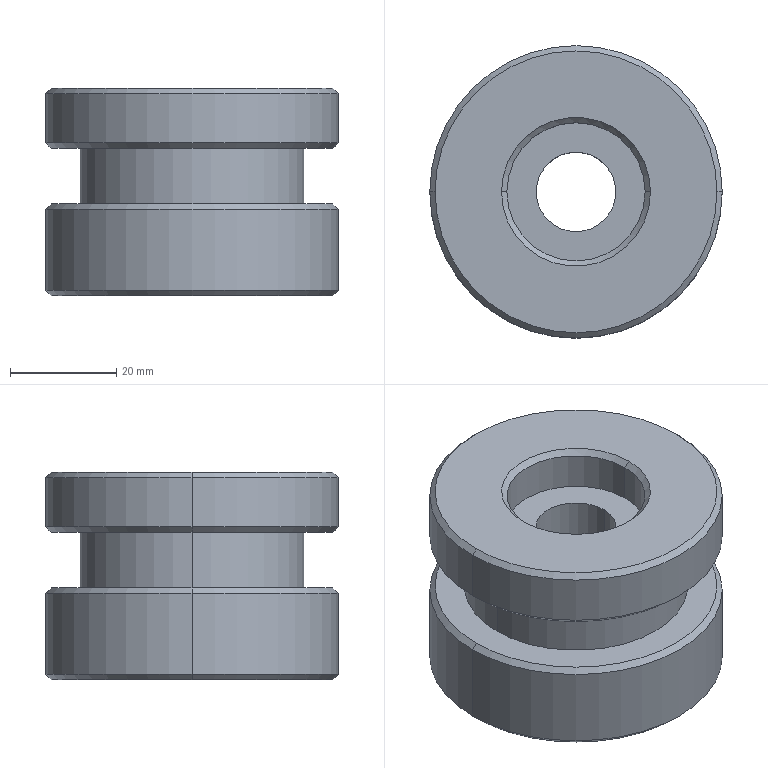Component | SolidWorks | 170423A4-PulleyAssembly-11_170423A4-Pulley1-1 | 1 solid | 30 faces | box 55 x 55 x 39 mm | volume 69274 mm3 | cone 12 | cylinder 12 | plane 6 | commonest cylinder face diameters 26 x4 55 x4 42 x2 15 x2
build123d program:
from build123d import *

# Parameters (mm, degrees)
SKETCH1_R           = 27.5
BOSS_EXTRUDE1_DEPTH = 19.5
SKETCH2_R           = 7.5
CUT_EXTRUDE1_DEPTH  = 56.077
SKETCH3_R           = 13
CUT_EXTRUDE2_DEPTH  = 8
CUT_EXTRUDE3_START  = -8
SKETCH4_R           = 13
CUT_EXTRUDE3_DEPTH  = 8
SKETCH5_W           = 6.5
SKETCH5_H           = 10.5
CHAMFER1_SIZE       = 1
CHAMFER2_SIZE       = 1


with BuildPart() as part:
    # Sketch1 → Boss-Extrude1 (new, symmetric)
    with BuildSketch(Plane.XY):
        Circle(SKETCH1_R)
    extrude(amount=BOSS_EXTRUDE1_DEPTH, both=True)

    # Sketch2 → Cut-Extrude1 (cut, through all)
    with BuildSketch(Plane.XY.offset(19.5)):
        Circle(SKETCH2_R)
    extrude(amount=-CUT_EXTRUDE1_DEPTH, mode=Mode.SUBTRACT)

    # Sketch3 → Cut-Extrude2 (cut)
    with BuildSketch(Plane.XY.offset(19.5)):
        Circle(SKETCH3_R)
    extrude(amount=-CUT_EXTRUDE2_DEPTH, mode=Mode.SUBTRACT)

    # Sketch4 → Cut-Extrude3 (cut)
    with BuildSketch(Plane(origin=(0, 0, -19.5), x_dir=(-1, 0, 0), z_dir=(0, 0, -1)).offset(CUT_EXTRUDE3_START)):
        with Locations(Location((0, 0, 0), (0, 0, 180))):
            Circle(SKETCH4_R)
    extrude(amount=CUT_EXTRUDE3_DEPTH, mode=Mode.SUBTRACT)

    # Sketch5 → Cut-Revolve1 (revolve, cut)
    with BuildSketch(Plane(origin=(0, 0, 0), x_dir=(1, 0, 0), z_dir=(0, 1, 0))):
        with Locations((-24.25, -3)):
            Rectangle(SKETCH5_W, SKETCH5_H)
    revolve(axis=Axis((0, 0, 0), (0, 0, 1)), mode=Mode.SUBTRACT)

    # Chamfer1
    chamfer1_edges = [part.edges().sort_by_distance(p)[0] for p in [
        (-27.5, 0, -19.5),
        (-27.5, 0, 8.25),
        (-27.5, 0, -2.25),
        (-27.5, 0, 19.5),
    ]]
    chamfer(chamfer1_edges, length=CHAMFER1_SIZE)

    # Chamfer2
    chamfer2_edges = [part.edges().sort_by_distance(p)[0] for p in [
        (-13, 0, 19.5),
        (-13, 0, -19.5),
    ]]
    chamfer(chamfer2_edges, length=CHAMFER2_SIZE)


solid = part.part

# Placed as in the assembly
solid = solid.moved(Location((139.754, -5.788, 441), (0, 0, 0)))
STEP:
#1=CARTESIAN_POINT('',(4.99,-0.2279,16.634));
#2=VERTEX_POINT('',#1);
#3=CARTESIAN_POINT('',(6.014,-0.2279,16.634));
#4=VERTEX_POINT('',#3);
#5=CARTESIAN_POINT('',(5.502,-0.2279,16.634));
#6=DIRECTION('',(0.,0.,-1.));
#7=DIRECTION('',(-1.,0.,0.));
#8=AXIS2_PLACEMENT_3D('',#5,#6,#7);
#9=CIRCLE('',#8,0.5118);
#10=EDGE_CURVE('',#2,#4,#9,.T.);
#11=ORIENTED_EDGE('',*,*,#10,.F.);
#12=CARTESIAN_POINT('',(4.951,-0.2279,16.594));
#13=VERTEX_POINT('',#12);
#14=CARTESIAN_POINT('',(4.99,-0.2279,16.634));
#15=DIRECTION('',(-0.7071,-0.,-0.7071));
#16=VECTOR('',#15,39.37);
#17=LINE('',#14,#16);
#18=EDGE_CURVE('',#2,#13,#17,.T.);
#19=ORIENTED_EDGE('',*,*,#18,.T.);
#20=CARTESIAN_POINT('',(6.053,-0.2279,16.594));
#21=VERTEX_POINT('',#20);
#22=CARTESIAN_POINT('',(5.502,-0.2279,16.594));
#23=DIRECTION('',(0.,0.,1.));
#24=DIRECTION('',(-1.,0.,0.));
#25=AXIS2_PLACEMENT_3D('',#22,#23,#24);
#26=CIRCLE('',#25,0.5512);
#27=EDGE_CURVE('',#21,#13,#26,.T.);
#28=ORIENTED_EDGE('',*,*,#27,.F.);
#29=CARTESIAN_POINT('',(6.014,-0.2279,16.634));
#30=DIRECTION('',(0.7071,0.,-0.7071));
#31=VECTOR('',#30,39.37);
#32=LINE('',#29,#31);
#33=EDGE_CURVE('',#4,#21,#32,.T.);
#34=ORIENTED_EDGE('',*,*,#33,.F.);
#35=EDGE_LOOP('',(#11,#19,#28,#34));
#36=FACE_OUTER_BOUND('',#35,.T.);
#37=CARTESIAN_POINT('',(5.502,-0.2279,16.634));
#38=DIRECTION('',(0.,0.,-1.));
#39=DIRECTION('',(1.,0.,0.));
#40=AXIS2_PLACEMENT_3D('',#37,#38,#39);
#41=CONICAL_SURFACE('',#40,0.5118,0.7854);
#42=ADVANCED_FACE('',(#36),#41,.F.);
#43=CARTESIAN_POINT('',(6.014,-0.2279,18.091));
#44=VERTEX_POINT('',#43);
#45=CARTESIAN_POINT('',(4.99,-0.2279,18.091));
#46=VERTEX_POINT('',#45);
#47=CARTESIAN_POINT('',(5.502,-0.2279,18.091));
#48=DIRECTION('',(0.,0.,1.));
#49=DIRECTION('',(-1.,0.,0.));
#50=AXIS2_PLACEMENT_3D('',#47,#48,#49);
#51=CIRCLE('',#50,0.5118);
#52=EDGE_CURVE('',#44,#46,#51,.T.);
#53=ORIENTED_EDGE('',*,*,#52,.F.);
#54=CARTESIAN_POINT('',(6.053,-0.2279,18.13));
#55=VERTEX_POINT('',#54);
#56=CARTESIAN_POINT('',(6.014,-0.2279,18.091));
#57=DIRECTION('',(0.7071,-0.,0.7071));
#58=VECTOR('',#57,39.37);
#59=LINE('',#56,#58);
#60=EDGE_CURVE('',#44,#55,#59,.T.);
#61=ORIENTED_EDGE('',*,*,#60,.T.);
#62=CARTESIAN_POINT('',(4.951,-0.2279,18.13));
#63=VERTEX_POINT('',#62);
#64=CARTESIAN_POINT('',(5.502,-0.2279,18.13));
#65=DIRECTION('',(0.,0.,-1.));
#66=DIRECTION('',(-1.,0.,0.));
#67=AXIS2_PLACEMENT_3D('',#64,#65,#66);
#68=CIRCLE('',#67,0.5512);
#69=EDGE_CURVE('',#63,#55,#68,.T.);
#70=ORIENTED_EDGE('',*,*,#69,.F.);
#71=CARTESIAN_POINT('',(4.99,-0.2279,18.091));
#72=DIRECTION('',(-0.7071,0.,0.7071));
#73=VECTOR('',#72,39.37);
#74=LINE('',#71,#73);
#75=EDGE_CURVE('',#46,#63,#74,.T.);
#76=ORIENTED_EDGE('',*,*,#75,.F.);
#77=EDGE_LOOP('',(#53,#61,#70,#76));
#78=FACE_OUTER_BOUND('',#77,.T.);
#79=CARTESIAN_POINT('',(5.502,-0.2279,18.091));
#80=DIRECTION('',(0.,0.,1.));
#81=DIRECTION('',(-1.,0.,0.));
#82=AXIS2_PLACEMENT_3D('',#79,#80,#81);
#83=CONICAL_SURFACE('',#82,0.5118,0.7854);
#84=ADVANCED_FACE('',(#78),#83,.F.);
#85=CARTESIAN_POINT('',(4.459,-0.2279,18.13));
#86=VERTEX_POINT('',#85);
#87=CARTESIAN_POINT('',(6.545,-0.2279,18.13));
#88=VERTEX_POINT('',#87);
#89=CARTESIAN_POINT('',(5.502,-0.2279,18.13));
#90=DIRECTION('',(0.,0.,1.));
#91=DIRECTION('',(-1.,0.,0.));
#92=AXIS2_PLACEMENT_3D('',#89,#90,#91);
#93=CIRCLE('',#92,1.043);
#94=EDGE_CURVE('',#86,#88,#93,.T.);
#95=ORIENTED_EDGE('',*,*,#94,.F.);
#96=CARTESIAN_POINT('',(4.419,-0.2279,18.091));
#97=VERTEX_POINT('',#96);
#98=CARTESIAN_POINT('',(4.459,-0.2279,18.13));
#99=DIRECTION('',(-0.7071,-0.,-0.7071));
#100=VECTOR('',#99,39.37);
#101=LINE('',#98,#100);
#102=EDGE_CURVE('',#86,#97,#101,.T.);
#103=ORIENTED_EDGE('',*,*,#102,.T.);
#104=CARTESIAN_POINT('',(6.585,-0.2279,18.091));
#105=VERTEX_POINT('',#104);
#106=CARTESIAN_POINT('',(5.502,-0.2279,18.091));
#107=DIRECTION('',(0.,0.,-1.));
#108=DIRECTION('',(-1.,0.,0.));
#109=AXIS2_PLACEMENT_3D('',#106,#107,#108);
#110=CIRCLE('',#109,1.083);
#111=EDGE_CURVE('',#105,#97,#110,.T.);
#112=ORIENTED_EDGE('',*,*,#111,.F.);
#113=CARTESIAN_POINT('',(6.545,-0.2279,18.13));
#114=DIRECTION('',(0.7071,0.,-0.7071));
#115=VECTOR('',#114,39.37);
#116=LINE('',#113,#115);
#117=EDGE_CURVE('',#88,#105,#116,.T.);
#118=ORIENTED_EDGE('',*,*,#117,.F.);
#119=EDGE_LOOP('',(#95,#103,#112,#118));
#120=FACE_OUTER_BOUND('',#119,.T.);
#121=CARTESIAN_POINT('',(5.502,-0.2279,18.13));
#122=DIRECTION('',(0.,0.,-1.));
#123=DIRECTION('',(1.,0.,0.));
#124=AXIS2_PLACEMENT_3D('',#121,#122,#123);
#125=CONICAL_SURFACE('',#124,1.043,0.7854);
#126=ADVANCED_FACE('',(#120),#125,.T.);
#127=CARTESIAN_POINT('',(6.545,-0.2279,17.687));
#128=VERTEX_POINT('',#127);
#129=CARTESIAN_POINT('',(4.459,-0.2279,17.687));
#130=VERTEX_POINT('',#129);
#131=CARTESIAN_POINT('',(5.502,-0.2279,17.687));
#132=DIRECTION('',(0.,0.,-1.));
#133=DIRECTION('',(-1.,0.,0.));
#134=AXIS2_PLACEMENT_3D('',#131,#132,#133);
#135=CIRCLE('',#134,1.043);
#136=EDGE_CURVE('',#128,#130,#135,.T.);
#137=ORIENTED_EDGE('',*,*,#136,.F.);
#138=CARTESIAN_POINT('',(6.585,-0.2279,17.726));
#139=VERTEX_POINT('',#138);
#140=CARTESIAN_POINT('',(6.545,-0.2279,17.687));
#141=DIRECTION('',(0.7071,-0.,0.7071));
#142=VECTOR('',#141,39.37);
#143=LINE('',#140,#142);
#144=EDGE_CURVE('',#128,#139,#143,.T.);
#145=ORIENTED_EDGE('',*,*,#144,.T.);
#146=CARTESIAN_POINT('',(4.419,-0.2279,17.726));
#147=VERTEX_POINT('',#146);
#148=CARTESIAN_POINT('',(5.502,-0.2279,17.726));
#149=DIRECTION('',(0.,0.,1.));
#150=DIRECTION('',(-1.,0.,0.));
#151=AXIS2_PLACEMENT_3D('',#148,#149,#150);
#152=CIRCLE('',#151,1.083);
#153=EDGE_CURVE('',#147,#139,#152,.T.);
#154=ORIENTED_EDGE('',*,*,#153,.F.);
#155=CARTESIAN_POINT('',(4.459,-0.2279,17.687));
#156=DIRECTION('',(-0.7071,0.,0.7071));
#157=VECTOR('',#156,39.37);
#158=LINE('',#155,#157);
#159=EDGE_CURVE('',#130,#147,#158,.T.);
#160=ORIENTED_EDGE('',*,*,#159,.F.);
#161=EDGE_LOOP('',(#137,#145,#154,#160));
#162=FACE_OUTER_BOUND('',#161,.T.);
#163=CARTESIAN_POINT('',(5.502,-0.2279,17.687));
#164=DIRECTION('',(0.,0.,1.));
#165=DIRECTION('',(-1.,0.,0.));
#166=AXIS2_PLACEMENT_3D('',#163,#164,#165);
#167=CONICAL_SURFACE('',#166,1.043,0.7854);
#168=ADVANCED_FACE('',(#162),#167,.T.);
#169=CARTESIAN_POINT('',(4.459,-0.2279,17.274));
#170=VERTEX_POINT('',#169);
#171=CARTESIAN_POINT('',(6.545,-0.2279,17.274));
#172=VERTEX_POINT('',#171);
#173=CARTESIAN_POINT('',(5.502,-0.2279,17.274));
#174=DIRECTION('',(-0.,0.,1.));
#175=DIRECTION('',(1.,0.,0.));
#176=AXIS2_PLACEMENT_3D('',#173,#174,#175);
#177=CIRCLE('',#176,1.043);
#178=EDGE_CURVE('',#170,#172,#177,.T.);
#179=ORIENTED_EDGE('',*,*,#178,.F.);
#180=CARTESIAN_POINT('',(4.419,-0.2279,17.234));
#181=VERTEX_POINT('',#180);
#182=CARTESIAN_POINT('',(4.419,-0.2279,17.234));
#183=DIRECTION('',(-0.7071,-0.,-0.7071));
#184=VECTOR('',#183,39.37);
#185=LINE('',#182,#184);
#186=EDGE_CURVE('',#170,#181,#185,.T.);
#187=ORIENTED_EDGE('',*,*,#186,.T.);
#188=CARTESIAN_POINT('',(6.585,-0.2279,17.234));
#189=VERTEX_POINT('',#188);
#190=CARTESIAN_POINT('',(5.502,-0.2279,17.234));
#191=DIRECTION('',(0.,0.,-1.));
#192=DIRECTION('',(1.,0.,0.));
#193=AXIS2_PLACEMENT_3D('',#190,#191,#192);
#194=CIRCLE('',#193,1.083);
#195=EDGE_CURVE('',#189,#181,#194,.T.);
#196=ORIENTED_EDGE('',*,*,#195,.F.);
#197=CARTESIAN_POINT('',(6.585,-0.2279,17.234));
#198=DIRECTION('',(0.7071,0.,-0.7071));
#199=VECTOR('',#198,39.37);
#200=LINE('',#197,#199);
#201=EDGE_CURVE('',#172,#189,#200,.T.);
#202=ORIENTED_EDGE('',*,*,#201,.F.);
#203=EDGE_LOOP('',(#179,#187,#196,#202));
#204=FACE_OUTER_BOUND('',#203,.T.);
#205=CARTESIAN_POINT('',(5.502,-0.2279,17.234));
#206=DIRECTION('',(0.,0.,-1.));
#207=DIRECTION('',(1.,0.,0.));
#208=AXIS2_PLACEMENT_3D('',#205,#206,#207);
#209=CONICAL_SURFACE('',#208,1.083,0.7854);
#210=ADVANCED_FACE('',(#204),#209,.T.);
#211=CARTESIAN_POINT('',(6.545,-0.2279,16.594));
#212=VERTEX_POINT('',#211);
#213=CARTESIAN_POINT('',(4.459,-0.2279,16.594));
#214=VERTEX_POINT('',#213);
#215=CARTESIAN_POINT('',(5.502,-0.2279,16.594));
#216=DIRECTION('',(0.,0.,-1.));
#217=DIRECTION('',(-1.,0.,0.));
#218=AXIS2_PLACEMENT_3D('',#215,#216,#217);
#219=CIRCLE('',#218,1.043);
#220=EDGE_CURVE('',#212,#214,#219,.T.);
#221=ORIENTED_EDGE('',*,*,#220,.F.);
#222=CARTESIAN_POINT('',(6.585,-0.2279,16.634));
#223=VERTEX_POINT('',#222);
#224=CARTESIAN_POINT('',(6.585,-0.2279,16.634));
#225=DIRECTION('',(0.7071,-0.,0.7071));
#226=VECTOR('',#225,39.37);
#227=LINE('',#224,#226);
#228=EDGE_CURVE('',#212,#223,#227,.T.);
#229=ORIENTED_EDGE('',*,*,#228,.T.);
#230=CARTESIAN_POINT('',(4.419,-0.2279,16.634));
#231=VERTEX_POINT('',#230);
#232=CARTESIAN_POINT('',(5.502,-0.2279,16.634));
#233=DIRECTION('',(0.,0.,1.));
#234=DIRECTION('',(-1.,0.,0.));
#235=AXIS2_PLACEMENT_3D('',#232,#233,#234);
#236=CIRCLE('',#235,1.083);
#237=EDGE_CURVE('',#231,#223,#236,.T.);
#238=ORIENTED_EDGE('',*,*,#237,.F.);
#239=CARTESIAN_POINT('',(4.419,-0.2279,16.634));
#240=DIRECTION('',(-0.7071,0.,0.7071));
#241=VECTOR('',#240,39.37);
#242=LINE('',#239,#241);
#243=EDGE_CURVE('',#214,#231,#242,.T.);
#244=ORIENTED_EDGE('',*,*,#243,.F.);
#245=EDGE_LOOP('',(#221,#229,#238,#244));
#246=FACE_OUTER_BOUND('',#245,.T.);
#247=CARTESIAN_POINT('',(5.502,-0.2279,16.634));
#248=DIRECTION('',(0.,0.,1.));
#249=DIRECTION('',(-1.,0.,0.));
#250=AXIS2_PLACEMENT_3D('',#247,#248,#249);
#251=CONICAL_SURFACE('',#250,1.083,0.7854);
#252=ADVANCED_FACE('',(#246),#251,.T.);
#253=CARTESIAN_POINT('',(6.329,-0.2279,17.687));
#254=VERTEX_POINT('',#253);
#255=CARTESIAN_POINT('',(4.675,-0.2279,17.687));
#256=VERTEX_POINT('',#255);
#257=CARTESIAN_POINT('',(5.502,-0.2279,17.687));
#258=DIRECTION('',(0.,0.,-1.));
#259=DIRECTION('',(1.,0.,0.));
#260=AXIS2_PLACEMENT_3D('',#257,#258,#259);
#261=CIRCLE('',#260,0.8268);
#262=EDGE_CURVE('',#254,#256,#261,.T.);
#263=ORIENTED_EDGE('',*,*,#262,.T.);
#264=CARTESIAN_POINT('',(4.675,-0.2279,17.274));
#265=VERTEX_POINT('',#264);
#266=CARTESIAN_POINT('',(4.675,-0.2279,17.362));
#267=DIRECTION('',(0.,0.,-1.));
#268=VECTOR('',#267,39.37);
#269=LINE('',#266,#268);
#270=EDGE_CURVE('',#256,#265,#269,.T.);
#271=ORIENTED_EDGE('',*,*,#270,.T.);
#272=CARTESIAN_POINT('',(6.329,-0.2279,17.274));
#273=VERTEX_POINT('',#272);
#274=CARTESIAN_POINT('',(5.502,-0.2279,17.274));
#275=DIRECTION('',(0.,0.,-1.));
#276=DIRECTION('',(1.,0.,0.));
#277=AXIS2_PLACEMENT_3D('',#274,#275,#276);
#278=CIRCLE('',#277,0.8268);
#279=EDGE_CURVE('',#273,#265,#278,.T.);
#280=ORIENTED_EDGE('',*,*,#279,.F.);
#281=CARTESIAN_POINT('',(6.329,-0.2279,17.362));
#282=DIRECTION('',(0.,0.,-1.));
#283=VECTOR('',#282,39.37);
#284=LINE('',#281,#283);
#285=EDGE_CURVE('',#254,#273,#284,.T.);
#286=ORIENTED_EDGE('',*,*,#285,.F.);
#287=EDGE_LOOP('',(#263,#271,#280,#286));
#288=FACE_OUTER_BOUND('',#287,.T.);
#289=CARTESIAN_POINT('',(5.502,-0.2279,17.362));
#290=DIRECTION('',(0.,0.,-1.));
#291=DIRECTION('',(1.,0.,0.));
#292=AXIS2_PLACEMENT_3D('',#289,#290,#291);
#293=CYLINDRICAL_SURFACE('',#292,0.8268);
#294=ADVANCED_FACE('',(#288),#293,.T.);
#295=CARTESIAN_POINT('',(4.99,-0.2279,16.909));
#296=VERTEX_POINT('',#295);
#297=CARTESIAN_POINT('',(6.014,-0.2279,16.909));
#298=VERTEX_POINT('',#297);
#299=CARTESIAN_POINT('',(5.502,-0.2279,16.909));
#300=DIRECTION('',(0.,0.,-1.));
#301=DIRECTION('',(1.,0.,0.));
#302=AXIS2_PLACEMENT_3D('',#299,#300,#301);
#303=CIRCLE('',#302,0.5118);
#304=EDGE_CURVE('',#296,#298,#303,.T.);
#305=ORIENTED_EDGE('',*,*,#304,.F.);
#306=CARTESIAN_POINT('',(4.99,-0.2279,16.909));
#307=DIRECTION('',(0.,0.,-1.));
#308=VECTOR('',#307,39.37);
#309=LINE('',#306,#308);
#310=EDGE_CURVE('',#296,#2,#309,.T.);
#311=ORIENTED_EDGE('',*,*,#310,.T.);
#312=ORIENTED_EDGE('',*,*,#10,.T.);
#313=CARTESIAN_POINT('',(6.014,-0.2279,16.909));
#314=DIRECTION('',(0.,0.,-1.));
#315=VECTOR('',#314,39.37);
#316=LINE('',#313,#315);
#317=EDGE_CURVE('',#298,#4,#316,.T.);
#318=ORIENTED_EDGE('',*,*,#317,.F.);
#319=EDGE_LOOP('',(#305,#311,#312,#318));
#320=FACE_OUTER_BOUND('',#319,.T.);
#321=CARTESIAN_POINT('',(5.502,-0.2279,16.909));
#322=DIRECTION('',(0.,0.,-1.));
#323=DIRECTION('',(1.,0.,0.));
#324=AXIS2_PLACEMENT_3D('',#321,#322,#323);
#325=CYLINDRICAL_SURFACE('',#324,0.5118);
#326=ADVANCED_FACE('',(#320),#325,.F.);
#327=CARTESIAN_POINT('',(6.014,-0.2279,17.815));
#328=VERTEX_POINT('',#327);
#329=CARTESIAN_POINT('',(4.99,-0.2279,17.815));
#330=VERTEX_POINT('',#329);
#331=CARTESIAN_POINT('',(5.502,-0.2279,17.815));
#332=DIRECTION('',(0.,0.,1.));
#333=DIRECTION('',(-1.,0.,0.));
#334=AXIS2_PLACEMENT_3D('',#331,#332,#333);
#335=CIRCLE('',#334,0.5118);
#336=EDGE_CURVE('',#328,#330,#335,.T.);
#337=ORIENTED_EDGE('',*,*,#336,.F.);
#338=CARTESIAN_POINT('',(6.014,-0.2279,17.815));
#339=DIRECTION('',(0.,0.,1.));
#340=VECTOR('',#339,39.37);
#341=LINE('',#338,#340);
#342=EDGE_CURVE('',#328,#44,#341,.T.);
#343=ORIENTED_EDGE('',*,*,#342,.T.);
#344=ORIENTED_EDGE('',*,*,#52,.T.);
#345=CARTESIAN_POINT('',(4.99,-0.2279,17.815));
#346=DIRECTION('',(0.,0.,1.));
#347=VECTOR('',#346,39.37);
#348=LINE('',#345,#347);
#349=EDGE_CURVE('',#330,#46,#348,.T.);
#350=ORIENTED_EDGE('',*,*,#349,.F.);
#351=EDGE_LOOP('',(#337,#343,#344,#350));
#352=FACE_OUTER_BOUND('',#351,.T.);
#353=CARTESIAN_POINT('',(5.502,-0.2279,17.815));
#354=DIRECTION('',(0.,0.,1.));
#355=DIRECTION('',(-1.,0.,0.));
#356=AXIS2_PLACEMENT_3D('',#353,#354,#355);
#357=CYLINDRICAL_SURFACE('',#356,0.5118);
#358=ADVANCED_FACE('',(#352),#357,.F.);
#359=ORIENTED_EDGE('',*,*,#195,.T.);
#360=CARTESIAN_POINT('',(4.419,-0.2279,18.13));
#361=DIRECTION('',(0.,0.,-1.));
#362=VECTOR('',#361,39.37);
#363=LINE('',#360,#362);
#364=EDGE_CURVE('',#181,#231,#363,.T.);
#365=ORIENTED_EDGE('',*,*,#364,.T.);
#366=ORIENTED_EDGE('',*,*,#237,.T.);
#367=CARTESIAN_POINT('',(6.585,-0.2279,18.13));
#368=DIRECTION('',(0.,0.,-1.));
#369=VECTOR('',#368,39.37);
#370=LINE('',#367,#369);
#371=EDGE_CURVE('',#189,#223,#370,.T.);
#372=ORIENTED_EDGE('',*,*,#371,.F.);
#373=EDGE_LOOP('',(#359,#365,#366,#372));
#374=FACE_OUTER_BOUND('',#373,.T.);
#375=CARTESIAN_POINT('',(5.502,-0.2279,18.13));
#376=DIRECTION('',(0.,0.,-1.));
#377=DIRECTION('',(1.,0.,0.));
#378=AXIS2_PLACEMENT_3D('',#375,#376,#377);
#379=CYLINDRICAL_SURFACE('',#378,1.083);
#380=ADVANCED_FACE('',(#374),#379,.T.);
#381=CARTESIAN_POINT('',(5.797,-0.2279,16.909));
#382=VERTEX_POINT('',#381);
#383=CARTESIAN_POINT('',(5.207,-0.2279,16.909));
#384=VERTEX_POINT('',#383);
#385=CARTESIAN_POINT('',(5.502,-0.2279,16.909));
#386=DIRECTION('',(0.,0.,1.));
#387=DIRECTION('',(1.,0.,0.));
#388=AXIS2_PLACEMENT_3D('',#385,#386,#387);
#389=CIRCLE('',#388,0.2953);
#390=EDGE_CURVE('',#382,#384,#389,.T.);
#391=ORIENTED_EDGE('',*,*,#390,.F.);
#392=CARTESIAN_POINT('',(5.797,-0.2279,17.815));
#393=VERTEX_POINT('',#392);
#394=CARTESIAN_POINT('',(5.797,-0.2279,16.594));
#395=DIRECTION('',(0.,0.,1.));
#396=VECTOR('',#395,39.37);
#397=LINE('',#394,#396);
#398=EDGE_CURVE('',#382,#393,#397,.T.);
#399=ORIENTED_EDGE('',*,*,#398,.T.);
#400=CARTESIAN_POINT('',(5.207,-0.2279,17.815));
#401=VERTEX_POINT('',#400);
#402=CARTESIAN_POINT('',(5.502,-0.2279,17.815));
#403=DIRECTION('',(0.,0.,-1.));
#404=DIRECTION('',(-1.,0.,0.));
#405=AXIS2_PLACEMENT_3D('',#402,#403,#404);
#406=CIRCLE('',#405,0.2953);
#407=EDGE_CURVE('',#401,#393,#406,.T.);
#408=ORIENTED_EDGE('',*,*,#407,.F.);
#409=CARTESIAN_POINT('',(5.207,-0.2279,16.594));
#410=DIRECTION('',(0.,0.,1.));
#411=VECTOR('',#410,39.37);
#412=LINE('',#409,#411);
#413=EDGE_CURVE('',#384,#401,#412,.T.);
#414=ORIENTED_EDGE('',*,*,#413,.F.);
#415=EDGE_LOOP('',(#391,#399,#408,#414));
#416=FACE_OUTER_BOUND('',#415,.T.);
#417=CARTESIAN_POINT('',(5.502,-0.2279,16.594));
#418=DIRECTION('',(0.,0.,1.));
#419=DIRECTION('',(-1.,0.,0.));
#420=AXIS2_PLACEMENT_3D('',#417,#418,#419);
#421=CYLINDRICAL_SURFACE('',#420,0.2953);
#422=ADVANCED_FACE('',(#416),#421,.F.);
#423=ORIENTED_EDGE('',*,*,#111,.T.);
#424=CARTESIAN_POINT('',(4.419,-0.2279,18.13));
#425=DIRECTION('',(0.,0.,-1.));
#426=VECTOR('',#425,39.37);
#427=LINE('',#424,#426);
#428=EDGE_CURVE('',#97,#147,#427,.T.);
#429=ORIENTED_EDGE('',*,*,#428,.T.);
#430=ORIENTED_EDGE('',*,*,#153,.T.);
#431=CARTESIAN_POINT('',(6.585,-0.2279,18.13));
#432=DIRECTION('',(0.,0.,-1.));
#433=VECTOR('',#432,39.37);
#434=LINE('',#431,#433);
#435=EDGE_CURVE('',#105,#139,#434,.T.);
#436=ORIENTED_EDGE('',*,*,#435,.F.);
#437=EDGE_LOOP('',(#423,#429,#430,#436));
#438=FACE_OUTER_BOUND('',#437,.T.);
#439=CARTESIAN_POINT('',(5.502,-0.2279,18.13));
#440=DIRECTION('',(0.,0.,-1.));
#441=DIRECTION('',(1.,0.,0.));
#442=AXIS2_PLACEMENT_3D('',#439,#440,#441);
#443=CYLINDRICAL_SURFACE('',#442,1.083);
#444=ADVANCED_FACE('',(#438),#443,.T.);
#445=ORIENTED_EDGE('',*,*,#428,.F.);
#446=CARTESIAN_POINT('',(5.502,-0.2279,18.091));
#447=DIRECTION('',(0.,0.,-1.));
#448=DIRECTION('',(-1.,0.,0.));
#449=AXIS2_PLACEMENT_3D('',#446,#447,#448);
#450=CIRCLE('',#449,1.083);
#451=EDGE_CURVE('',#97,#105,#450,.T.);
#452=ORIENTED_EDGE('',*,*,#451,.T.);
#453=ORIENTED_EDGE('',*,*,#435,.T.);
#454=CARTESIAN_POINT('',(5.502,-0.2279,17.726));
#455=DIRECTION('',(0.,0.,1.));
#456=DIRECTION('',(-1.,0.,0.));
#457=AXIS2_PLACEMENT_3D('',#454,#455,#456);
#458=CIRCLE('',#457,1.083);
#459=EDGE_CURVE('',#139,#147,#458,.T.);
#460=ORIENTED_EDGE('',*,*,#459,.T.);
#461=EDGE_LOOP('',(#445,#452,#453,#460));
#462=FACE_OUTER_BOUND('',#461,.T.);
#463=CARTESIAN_POINT('',(5.502,-0.2279,18.13));
#464=DIRECTION('',(0.,0.,-1.));
#465=DIRECTION('',(1.,0.,0.));
#466=AXIS2_PLACEMENT_3D('',#463,#464,#465);
#467=CYLINDRICAL_SURFACE('',#466,1.083);
#468=ADVANCED_FACE('',(#462),#467,.T.);
#469=ORIENTED_EDGE('',*,*,#398,.F.);
#470=CARTESIAN_POINT('',(5.502,-0.2279,16.909));
#471=DIRECTION('',(0.,0.,1.));
#472=DIRECTION('',(1.,0.,0.));
#473=AXIS2_PLACEMENT_3D('',#470,#471,#472);
#474=CIRCLE('',#473,0.2953);
#475=EDGE_CURVE('',#384,#382,#474,.T.);
#476=ORIENTED_EDGE('',*,*,#475,.F.);
#477=ORIENTED_EDGE('',*,*,#413,.T.);
#478=CARTESIAN_POINT('',(5.502,-0.2279,17.815));
#479=DIRECTION('',(0.,0.,-1.));
#480=DIRECTION('',(-1.,0.,0.));
#481=AXIS2_PLACEMENT_3D('',#478,#479,#480);
#482=CIRCLE('',#481,0.2953);
#483=EDGE_CURVE('',#393,#401,#482,.T.);
#484=ORIENTED_EDGE('',*,*,#483,.F.);
#485=EDGE_LOOP('',(#469,#476,#477,#484));
#486=FACE_OUTER_BOUND('',#485,.T.);
#487=CARTESIAN_POINT('',(5.502,-0.2279,16.594));
#488=DIRECTION('',(0.,0.,1.));
#489=DIRECTION('',(-1.,0.,0.));
#490=AXIS2_PLACEMENT_3D('',#487,#488,#489);
#491=CYLINDRICAL_SURFACE('',#490,0.2953);
#492=ADVANCED_FACE('',(#486),#491,.F.);
#493=ORIENTED_EDGE('',*,*,#364,.F.);
#494=CARTESIAN_POINT('',(5.502,-0.2279,17.234));
#495=DIRECTION('',(0.,0.,-1.));
#496=DIRECTION('',(1.,0.,0.));
#497=AXIS2_PLACEMENT_3D('',#494,#495,#496);
#498=CIRCLE('',#497,1.083);
#499=EDGE_CURVE('',#181,#189,#498,.T.);
#500=ORIENTED_EDGE('',*,*,#499,.T.);
#501=ORIENTED_EDGE('',*,*,#371,.T.);
#502=CARTESIAN_POINT('',(5.502,-0.2279,16.634));
#503=DIRECTION('',(0.,0.,1.));
#504=DIRECTION('',(-1.,0.,0.));
#505=AXIS2_PLACEMENT_3D('',#502,#503,#504);
#506=CIRCLE('',#505,1.083);
#507=EDGE_CURVE('',#223,#231,#506,.T.);
#508=ORIENTED_EDGE('',*,*,#507,.T.);
#509=EDGE_LOOP('',(#493,#500,#501,#508));
#510=FACE_OUTER_BOUND('',#509,.T.);
#511=CARTESIAN_POINT('',(5.502,-0.2279,18.13));
#512=DIRECTION('',(0.,0.,-1.));
#513=DIRECTION('',(1.,0.,0.));
#514=AXIS2_PLACEMENT_3D('',#511,#512,#513);
#515=CYLINDRICAL_SURFACE('',#514,1.083);
#516=ADVANCED_FACE('',(#510),#515,.T.);
#517=ORIENTED_EDGE('',*,*,#69,.T.);
#518=CARTESIAN_POINT('',(5.502,-0.2279,18.13));
#519=DIRECTION('',(0.,0.,-1.));
#520=DIRECTION('',(-1.,0.,0.));
#521=AXIS2_PLACEMENT_3D('',#518,#519,#520);
#522=CIRCLE('',#521,0.5512);
#523=EDGE_CURVE('',#55,#63,#522,.T.);
#524=ORIENTED_EDGE('',*,*,#523,.T.);
#525=EDGE_LOOP('',(#517,#524));
#526=FACE_BOUND('',#525,.T.);
#527=CARTESIAN_POINT('',(5.502,-0.2279,18.13));
#528=DIRECTION('',(0.,0.,1.));
#529=DIRECTION('',(-1.,0.,0.));
#530=AXIS2_PLACEMENT_3D('',#527,#528,#529);
#531=CIRCLE('',#530,1.043);
#532=EDGE_CURVE('',#88,#86,#531,.T.);
#533=ORIENTED_EDGE('',*,*,#532,.T.);
#534=ORIENTED_EDGE('',*,*,#94,.T.);
#535=EDGE_LOOP('',(#533,#534));
#536=FACE_OUTER_BOUND('',#535,.T.);
#537=CARTESIAN_POINT('',(5.502,-0.2279,18.13));
#538=DIRECTION('',(0.,0.,1.));
#539=DIRECTION('',(-1.,0.,0.));
#540=AXIS2_PLACEMENT_3D('',#537,#538,#539);
#541=PLANE('',#540);
#542=ADVANCED_FACE('',(#526,#536),#541,.T.);
#543=ORIENTED_EDGE('',*,*,#27,.T.);
#544=CARTESIAN_POINT('',(5.502,-0.2279,16.594));
#545=DIRECTION('',(0.,0.,1.));
#546=DIRECTION('',(-1.,0.,0.));
#547=AXIS2_PLACEMENT_3D('',#544,#545,#546);
#548=CIRCLE('',#547,0.5512);
#549=EDGE_CURVE('',#13,#21,#548,.T.);
#550=ORIENTED_EDGE('',*,*,#549,.T.);
#551=EDGE_LOOP('',(#543,#550));
#552=FACE_BOUND('',#551,.T.);
#553=CARTESIAN_POINT('',(5.502,-0.2279,16.594));
#554=DIRECTION('',(0.,0.,-1.));
#555=DIRECTION('',(-1.,0.,0.));
#556=AXIS2_PLACEMENT_3D('',#553,#554,#555);
#557=CIRCLE('',#556,1.043);
#558=EDGE_CURVE('',#214,#212,#557,.T.);
#559=ORIENTED_EDGE('',*,*,#558,.T.);
#560=ORIENTED_EDGE('',*,*,#220,.T.);
#561=EDGE_LOOP('',(#559,#560));
#562=FACE_OUTER_BOUND('',#561,.T.);
#563=CARTESIAN_POINT('',(5.502,-0.2279,16.594));
#564=DIRECTION('',(0.,0.,1.));
#565=DIRECTION('',(-1.,0.,0.));
#566=AXIS2_PLACEMENT_3D('',#563,#564,#565);
#567=PLANE('',#566);
#568=ADVANCED_FACE('',(#552,#562),#567,.F.);
#569=CARTESIAN_POINT('',(5.502,-0.2279,17.815));
#570=DIRECTION('',(0.,0.,1.));
#571=DIRECTION('',(-1.,0.,0.));
#572=AXIS2_PLACEMENT_3D('',#569,#570,#571);
#573=CIRCLE('',#572,0.5118);
#574=EDGE_CURVE('',#330,#328,#573,.T.);
#575=ORIENTED_EDGE('',*,*,#574,.T.);
#576=ORIENTED_EDGE('',*,*,#336,.T.);
#577=EDGE_LOOP('',(#575,#576));
#578=FACE_OUTER_BOUND('',#577,.T.);
#579=ORIENTED_EDGE('',*,*,#407,.T.);
#580=ORIENTED_EDGE('',*,*,#483,.T.);
#581=EDGE_LOOP('',(#579,#580));
#582=FACE_BOUND('',#581,.T.);
#583=CARTESIAN_POINT('',(5.502,-0.2279,17.815));
#584=DIRECTION('',(0.,0.,1.));
#585=DIRECTION('',(-1.,0.,0.));
#586=AXIS2_PLACEMENT_3D('',#583,#584,#585);
#587=PLANE('',#586);
#588=ADVANCED_FACE('',(#578,#582),#587,.T.);
#589=ORIENTED_EDGE('',*,*,#342,.F.);
#590=ORIENTED_EDGE('',*,*,#574,.F.);
#591=ORIENTED_EDGE('',*,*,#349,.T.);
#592=CARTESIAN_POINT('',(5.502,-0.2279,18.091));
#593=DIRECTION('',(0.,0.,1.));
#594=DIRECTION('',(-1.,0.,0.));
#595=AXIS2_PLACEMENT_3D('',#592,#593,#594);
#596=CIRCLE('',#595,0.5118);
#597=EDGE_CURVE('',#46,#44,#596,.T.);
#598=ORIENTED_EDGE('',*,*,#597,.T.);
#599=EDGE_LOOP('',(#589,#590,#591,#598));
#600=FACE_OUTER_BOUND('',#599,.T.);
#601=CARTESIAN_POINT('',(5.502,-0.2279,17.815));
#602=DIRECTION('',(0.,0.,1.));
#603=DIRECTION('',(-1.,0.,0.));
#604=AXIS2_PLACEMENT_3D('',#601,#602,#603);
#605=CYLINDRICAL_SURFACE('',#604,0.5118);
#606=ADVANCED_FACE('',(#600),#605,.F.);
#607=CARTESIAN_POINT('',(5.502,-0.2279,16.909));
#608=DIRECTION('',(0.,0.,-1.));
#609=DIRECTION('',(1.,0.,0.));
#610=AXIS2_PLACEMENT_3D('',#607,#608,#609);
#611=CIRCLE('',#610,0.5118);
#612=EDGE_CURVE('',#298,#296,#611,.T.);
#613=ORIENTED_EDGE('',*,*,#612,.T.);
#614=ORIENTED_EDGE('',*,*,#304,.T.);
#615=EDGE_LOOP('',(#613,#614));
#616=FACE_OUTER_BOUND('',#615,.T.);
#617=ORIENTED_EDGE('',*,*,#475,.T.);
#618=ORIENTED_EDGE('',*,*,#390,.T.);
#619=EDGE_LOOP('',(#617,#618));
#620=FACE_BOUND('',#619,.T.);
#621=CARTESIAN_POINT('',(5.502,-0.2279,16.909));
#622=DIRECTION('',(0.,0.,-1.));
#623=DIRECTION('',(1.,0.,0.));
#624=AXIS2_PLACEMENT_3D('',#621,#622,#623);
#625=PLANE('',#624);
#626=ADVANCED_FACE('',(#616,#620),#625,.T.);
#627=ORIENTED_EDGE('',*,*,#310,.F.);
#628=ORIENTED_EDGE('',*,*,#612,.F.);
#629=ORIENTED_EDGE('',*,*,#317,.T.);
#630=CARTESIAN_POINT('',(5.502,-0.2279,16.634));
#631=DIRECTION('',(0.,0.,-1.));
#632=DIRECTION('',(-1.,0.,0.));
#633=AXIS2_PLACEMENT_3D('',#630,#631,#632);
#634=CIRCLE('',#633,0.5118);
#635=EDGE_CURVE('',#4,#2,#634,.T.);
#636=ORIENTED_EDGE('',*,*,#635,.T.);
#637=EDGE_LOOP('',(#627,#628,#629,#636));
#638=FACE_OUTER_BOUND('',#637,.T.);
#639=CARTESIAN_POINT('',(5.502,-0.2279,16.909));
#640=DIRECTION('',(0.,0.,-1.));
#641=DIRECTION('',(1.,0.,0.));
#642=AXIS2_PLACEMENT_3D('',#639,#640,#641);
#643=CYLINDRICAL_SURFACE('',#642,0.5118);
#644=ADVANCED_FACE('',(#638),#643,.F.);
#645=CARTESIAN_POINT('',(5.502,-0.2279,17.687));
#646=DIRECTION('',(0.,0.,-1.));
#647=DIRECTION('',(-1.,0.,0.));
#648=AXIS2_PLACEMENT_3D('',#645,#646,#647);
#649=CIRCLE('',#648,1.043);
#650=EDGE_CURVE('',#130,#128,#649,.T.);
#651=ORIENTED_EDGE('',*,*,#650,.T.);
#652=ORIENTED_EDGE('',*,*,#136,.T.);
#653=EDGE_LOOP('',(#651,#652));
#654=FACE_OUTER_BOUND('',#653,.T.);
#655=ORIENTED_EDGE('',*,*,#262,.F.);
#656=CARTESIAN_POINT('',(5.502,-0.2279,17.687));
#657=DIRECTION('',(0.,0.,-1.));
#658=DIRECTION('',(1.,0.,0.));
#659=AXIS2_PLACEMENT_3D('',#656,#657,#658);
#660=CIRCLE('',#659,0.8268);
#661=EDGE_CURVE('',#256,#254,#660,.T.);
#662=ORIENTED_EDGE('',*,*,#661,.F.);
#663=EDGE_LOOP('',(#655,#662));
#664=FACE_BOUND('',#663,.T.);
#665=CARTESIAN_POINT('',(6.585,-0.2279,17.687));
#666=DIRECTION('',(-0.,0.,1.));
#667=DIRECTION('',(-1.,0.,-0.));
#668=AXIS2_PLACEMENT_3D('',#665,#666,#667);
#669=PLANE('',#668);
#670=ADVANCED_FACE('',(#654,#664),#669,.F.);
#671=ORIENTED_EDGE('',*,*,#270,.F.);
#672=ORIENTED_EDGE('',*,*,#661,.T.);
#673=ORIENTED_EDGE('',*,*,#285,.T.);
#674=CARTESIAN_POINT('',(5.502,-0.2279,17.274));
#675=DIRECTION('',(0.,0.,-1.));
#676=DIRECTION('',(1.,0.,0.));
#677=AXIS2_PLACEMENT_3D('',#674,#675,#676);
#678=CIRCLE('',#677,0.8268);
#679=EDGE_CURVE('',#265,#273,#678,.T.);
#680=ORIENTED_EDGE('',*,*,#679,.F.);
#681=EDGE_LOOP('',(#671,#672,#673,#680));
#682=FACE_OUTER_BOUND('',#681,.T.);
#683=CARTESIAN_POINT('',(5.502,-0.2279,17.362));
#684=DIRECTION('',(0.,0.,-1.));
#685=DIRECTION('',(1.,0.,0.));
#686=AXIS2_PLACEMENT_3D('',#683,#684,#685);
#687=CYLINDRICAL_SURFACE('',#686,0.8268);
#688=ADVANCED_FACE('',(#682),#687,.T.);
#689=CARTESIAN_POINT('',(5.502,-0.2279,17.274));
#690=DIRECTION('',(-0.,0.,1.));
#691=DIRECTION('',(1.,0.,0.));
#692=AXIS2_PLACEMENT_3D('',#689,#690,#691);
#693=CIRCLE('',#692,1.043);
#694=EDGE_CURVE('',#172,#170,#693,.T.);
#695=ORIENTED_EDGE('',*,*,#694,.T.);
#696=ORIENTED_EDGE('',*,*,#178,.T.);
#697=EDGE_LOOP('',(#695,#696));
#698=FACE_OUTER_BOUND('',#697,.T.);
#699=ORIENTED_EDGE('',*,*,#279,.T.);
#700=ORIENTED_EDGE('',*,*,#679,.T.);
#701=EDGE_LOOP('',(#699,#700));
#702=FACE_BOUND('',#701,.T.);
#703=CARTESIAN_POINT('',(6.585,-0.2279,17.274));
#704=DIRECTION('',(0.,0.,-1.));
#705=DIRECTION('',(1.,0.,0.));
#706=AXIS2_PLACEMENT_3D('',#703,#704,#705);
#707=PLANE('',#706);
#708=ADVANCED_FACE('',(#698,#702),#707,.F.);
#709=ORIENTED_EDGE('',*,*,#228,.F.);
#710=ORIENTED_EDGE('',*,*,#558,.F.);
#711=ORIENTED_EDGE('',*,*,#243,.T.);
#712=ORIENTED_EDGE('',*,*,#507,.F.);
#713=EDGE_LOOP('',(#709,#710,#711,#712));
#714=FACE_OUTER_BOUND('',#713,.T.);
#715=CARTESIAN_POINT('',(5.502,-0.2279,16.634));
#716=DIRECTION('',(0.,0.,1.));
#717=DIRECTION('',(-1.,0.,0.));
#718=AXIS2_PLACEMENT_3D('',#715,#716,#717);
#719=CONICAL_SURFACE('',#718,1.083,0.7854);
#720=ADVANCED_FACE('',(#714),#719,.T.);
#721=ORIENTED_EDGE('',*,*,#186,.F.);
#722=ORIENTED_EDGE('',*,*,#694,.F.);
#723=ORIENTED_EDGE('',*,*,#201,.T.);
#724=ORIENTED_EDGE('',*,*,#499,.F.);
#725=EDGE_LOOP('',(#721,#722,#723,#724));
#726=FACE_OUTER_BOUND('',#725,.T.);
#727=CARTESIAN_POINT('',(5.502,-0.2279,17.234));
#728=DIRECTION('',(0.,0.,-1.));
#729=DIRECTION('',(1.,0.,0.));
#730=AXIS2_PLACEMENT_3D('',#727,#728,#729);
#731=CONICAL_SURFACE('',#730,1.083,0.7854);
#732=ADVANCED_FACE('',(#726),#731,.T.);
#733=ORIENTED_EDGE('',*,*,#144,.F.);
#734=ORIENTED_EDGE('',*,*,#650,.F.);
#735=ORIENTED_EDGE('',*,*,#159,.T.);
#736=ORIENTED_EDGE('',*,*,#459,.F.);
#737=EDGE_LOOP('',(#733,#734,#735,#736));
#738=FACE_OUTER_BOUND('',#737,.T.);
#739=CARTESIAN_POINT('',(5.502,-0.2279,17.687));
#740=DIRECTION('',(0.,0.,1.));
#741=DIRECTION('',(-1.,0.,0.));
#742=AXIS2_PLACEMENT_3D('',#739,#740,#741);
#743=CONICAL_SURFACE('',#742,1.043,0.7854);
#744=ADVANCED_FACE('',(#738),#743,.T.);
#745=ORIENTED_EDGE('',*,*,#102,.F.);
#746=ORIENTED_EDGE('',*,*,#532,.F.);
#747=ORIENTED_EDGE('',*,*,#117,.T.);
#748=ORIENTED_EDGE('',*,*,#451,.F.);
#749=EDGE_LOOP('',(#745,#746,#747,#748));
#750=FACE_OUTER_BOUND('',#749,.T.);
#751=CARTESIAN_POINT('',(5.502,-0.2279,18.13));
#752=DIRECTION('',(0.,0.,-1.));
#753=DIRECTION('',(1.,0.,0.));
#754=AXIS2_PLACEMENT_3D('',#751,#752,#753);
#755=CONICAL_SURFACE('',#754,1.043,0.7854);
#756=ADVANCED_FACE('',(#750),#755,.T.);
#757=ORIENTED_EDGE('',*,*,#60,.F.);
#758=ORIENTED_EDGE('',*,*,#597,.F.);
#759=ORIENTED_EDGE('',*,*,#75,.T.);
#760=ORIENTED_EDGE('',*,*,#523,.F.);
#761=EDGE_LOOP('',(#757,#758,#759,#760));
#762=FACE_OUTER_BOUND('',#761,.T.);
#763=CARTESIAN_POINT('',(5.502,-0.2279,18.091));
#764=DIRECTION('',(0.,0.,1.));
#765=DIRECTION('',(-1.,0.,0.));
#766=AXIS2_PLACEMENT_3D('',#763,#764,#765);
#767=CONICAL_SURFACE('',#766,0.5118,0.7854);
#768=ADVANCED_FACE('',(#762),#767,.F.);
#769=ORIENTED_EDGE('',*,*,#18,.F.);
#770=ORIENTED_EDGE('',*,*,#635,.F.);
#771=ORIENTED_EDGE('',*,*,#33,.T.);
#772=ORIENTED_EDGE('',*,*,#549,.F.);
#773=EDGE_LOOP('',(#769,#770,#771,#772));
#774=FACE_OUTER_BOUND('',#773,.T.);
#775=CARTESIAN_POINT('',(5.502,-0.2279,16.634));
#776=DIRECTION('',(0.,0.,-1.));
#777=DIRECTION('',(1.,0.,0.));
#778=AXIS2_PLACEMENT_3D('',#775,#776,#777);
#779=CONICAL_SURFACE('',#778,0.5118,0.7854);
#780=ADVANCED_FACE('',(#774),#779,.F.);
#781=CLOSED_SHELL('',(#42,#84,#126,#168,#210,#252,#294,#326,#358,#380,#422,#444,#468,#492,#516,#542,#568,#588,#606,#626,#644,#670,#688,#708,#720,#732,#744,#756,#768,#780));
#782=MANIFOLD_SOLID_BREP('',#781);
#783=CARTESIAN_POINT('',(0.,0.,0.));
#784=DIRECTION('',(0.,0.,1.));
#785=DIRECTION('',(1.,0.,0.));
#786=AXIS2_PLACEMENT_3D('',#783,#784,#785);
#787=(LENGTH_UNIT()NAMED_UNIT(*)SI_UNIT($,.METRE.));
#788=LENGTH_MEASURE_WITH_UNIT(LENGTH_MEASURE(0.0254),#787);
#789=DIMENSIONAL_EXPONENTS(1.,0.,0.,0.,0.,0.,0.);
#790=(CONVERSION_BASED_UNIT('',#788)LENGTH_UNIT()NAMED_UNIT(#789));
#791=UNCERTAINTY_MEASURE_WITH_UNIT(LENGTH_MEASURE(0.00001),#790,'','');
#792=(NAMED_UNIT(*)PLANE_ANGLE_UNIT()SI_UNIT($,.RADIAN.));
#793=(NAMED_UNIT(*)SI_UNIT($,.STERADIAN.)SOLID_ANGLE_UNIT());
#794=(GEOMETRIC_REPRESENTATION_CONTEXT(3)GLOBAL_UNCERTAINTY_ASSIGNED_CONTEXT((#791))GLOBAL_UNIT_ASSIGNED_CONTEXT((#790,#792,#793))REPRESENTATION_CONTEXT('',''));
#795=ADVANCED_BREP_SHAPE_REPRESENTATION('',(#782,#786),#794);
#796=COLOUR_RGB('',0.7922,0.8196,0.9333);
#797=FILL_AREA_STYLE_COLOUR('',#796);
#798=FILL_AREA_STYLE('',(#797));
#799=SURFACE_STYLE_FILL_AREA(#798);
#800=SURFACE_SIDE_STYLE('',(#799));
#801=SURFACE_STYLE_USAGE(.BOTH.,#800);
#802=PRESENTATION_STYLE_ASSIGNMENT((#801));
#803=STYLED_ITEM('',(#802),#782);
#804=PRESENTATION_LAYER_ASSIGNMENT('','',(#803));
#805=(LENGTH_UNIT()NAMED_UNIT(*)SI_UNIT($,.METRE.));
#806=LENGTH_MEASURE_WITH_UNIT(LENGTH_MEASURE(0.0254),#805);
#807=DIMENSIONAL_EXPONENTS(1.,0.,0.,0.,0.,0.,0.);
#808=(CONVERSION_BASED_UNIT('',#806)LENGTH_UNIT()NAMED_UNIT(#807));
#809=UNCERTAINTY_MEASURE_WITH_UNIT(LENGTH_MEASURE(0.00001),#808,'','');
#810=(NAMED_UNIT(*)PLANE_ANGLE_UNIT()SI_UNIT($,.RADIAN.));
#811=(NAMED_UNIT(*)SI_UNIT($,.STERADIAN.)SOLID_ANGLE_UNIT());
#812=(GEOMETRIC_REPRESENTATION_CONTEXT(3)GLOBAL_UNCERTAINTY_ASSIGNED_CONTEXT((#809))GLOBAL_UNIT_ASSIGNED_CONTEXT((#808,#810,#811))REPRESENTATION_CONTEXT('',''));
#813=MECHANICAL_DESIGN_GEOMETRIC_PRESENTATION_REPRESENTATION('',(#803),#812);